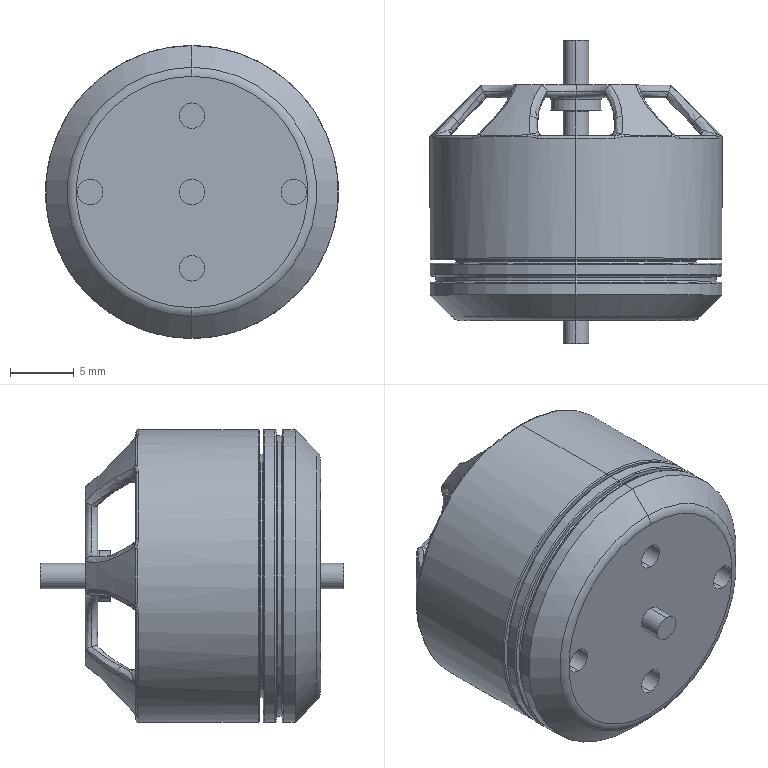Component | SolidWorks | 10.Motor-1 | 1 solid | 206 faces | box 23 x 23.8 x 23 mm | volume 5901 mm3 | spline 96 | torus 51 | cylinder 28 | plane 21 | cone 10 | commonest cylinder face diameters 2 x14 23 x6 4 x2 21 x2 19 x2 22 x2